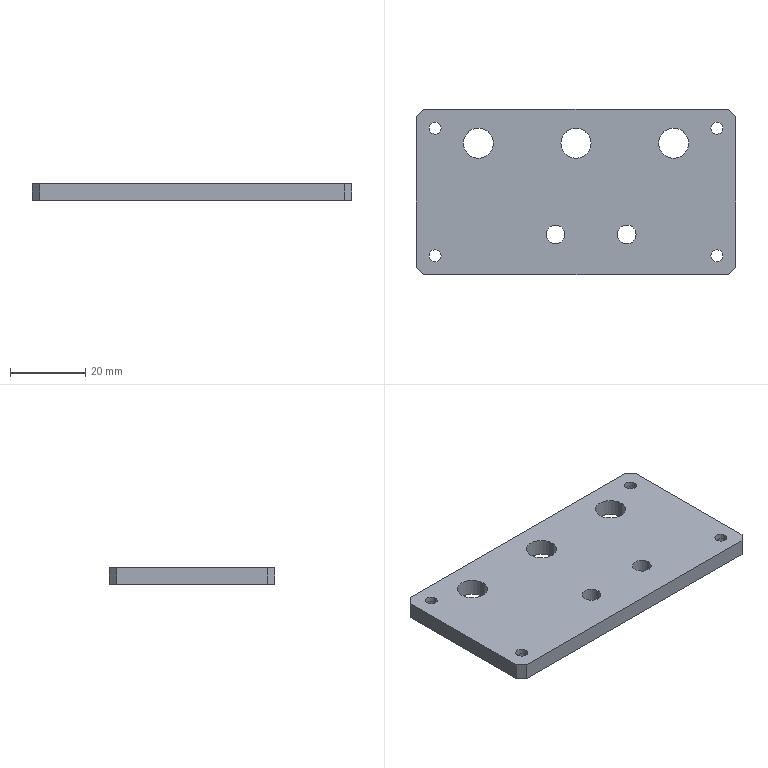Component | SolidWorks | 170423A4-SafetyPowerProbeProtectionPlate-1 | 1 solid | 40 faces | box 85 x 44 x 4.5 mm | volume 15429 mm3 | cylinder 26 | plane 14 | commonest cylinder face diameters 7 x8 3.2 x8 8 x6 5 x4
build123d program:
from build123d import *

# Parameters (mm, degrees)
SKETCH2_W                                       = 110
SKETCH2_H                                       = 50
BOSS_EXTRUDE1_DEPTH                             = 4.5
F_3_0_3_DIAMETER_HOLE1_D                        = 3
F_1_65_1_65_DIAMETER_HOLE1_D                    = 1.65
M3_HEX_SOCKET_HEAD_CAP_SCREW_CBORE2_D           = 3.2
M3_HEX_SOCKET_HEAD_CAP_SCREW_CBORE2_CBORE_D     = 7
M3_HEX_SOCKET_HEAD_CAP_SCREW_CBORE2_CBORE_DEPTH = 3
SKETCH13_R                                      = 4
SKETCH13_R_2                                    = 2.5
CUT_EXTRUDE1_DEPTH                              = 111.774
SKETCH14_W                                      = 110
SKETCH14_H                                      = 50
SKETCH14_W_2                                    = 85
SKETCH14_H_2                                    = 44
CUT_EXTRUDE2_DEPTH                              = 111.774
CHAMFER1_SIZE                                   = 2


with BuildPart() as part:
    # Sketch2 → Boss-Extrude1 (new body)
    with BuildSketch(Plane.XY):
        with Locations((37.907, 35.158)):
            Rectangle(SKETCH2_W, SKETCH2_H)
    extrude(amount=BOSS_EXTRUDE1_DEPTH)

    # 3.0 _3_ Diameter Hole1 (through all)
    with Locations(Plane.XY.offset(4.5)):
        with Locations((11.907, 48.158), (37.907, 48.158), (63.907, 48.158)):
            Hole(F_3_0_3_DIAMETER_HOLE1_D / 2)

    # 1.65 _1.65_ Diameter Hole1 (through all)
    with Locations(Plane.XY.offset(4.5)):
        with Locations((24.407, 23.874), (43.359, 23.874)):
            Hole(F_1_65_1_65_DIAMETER_HOLE1_D / 2)

    # M3 Hex Socket Head Cap Screw CBORE2 (through all)
    with Locations(Plane.XY.offset(4.5)):
        with Locations((0.4069, 52.158), (0.4069, 18.158), (75.407, 52.158), (75.407, 18.158)):
            CounterBoreHole(M3_HEX_SOCKET_HEAD_CAP_SCREW_CBORE2_D / 2, M3_HEX_SOCKET_HEAD_CAP_SCREW_CBORE2_CBORE_D / 2, M3_HEX_SOCKET_HEAD_CAP_SCREW_CBORE2_CBORE_DEPTH)

    # Sketch13 → Cut-Extrude1 (cut, through all)
    with BuildSketch(Plane.XY.offset(4.5)):
        with Locations((11.907, 48.158)):
            Circle(SKETCH13_R)
        with Locations((37.907, 48.158)):
            Circle(SKETCH13_R)
        with Locations((63.907, 48.158)):
            Circle(SKETCH13_R)
        with Locations((24.407, 23.874)):
            Circle(SKETCH13_R_2)
        with Locations((43.359, 23.874)):
            Circle(SKETCH13_R_2)
    extrude(amount=-CUT_EXTRUDE1_DEPTH, mode=Mode.SUBTRACT)

    # Sketch14 → Cut-Extrude2 (cut, through all)
    with BuildSketch(Plane.XY.offset(4.5)):
        with Locations((37.907, 35.158)):
            Rectangle(SKETCH14_W, SKETCH14_H)
        with Locations((37.907, 35.158)):
            Rectangle(SKETCH14_W_2, SKETCH14_H_2, mode=Mode.SUBTRACT)
    extrude(amount=-CUT_EXTRUDE2_DEPTH, mode=Mode.SUBTRACT)

    # Chamfer1
    chamfer1_edges = [part.edges().sort_by_distance(p)[0] for p in [
        (-4.593, 57.158, 2.25),
        (80.407, 57.158, 2.25),
        (80.407, 13.158, 2.25),
        (-4.593, 13.158, 2.25),
    ]]
    chamfer(chamfer1_edges, length=CHAMFER1_SIZE)


solid = part.part

# Placed as in the assembly
solid = solid.moved(Location((66.593, -20.769, -90.074), (-180, 0, 180)))